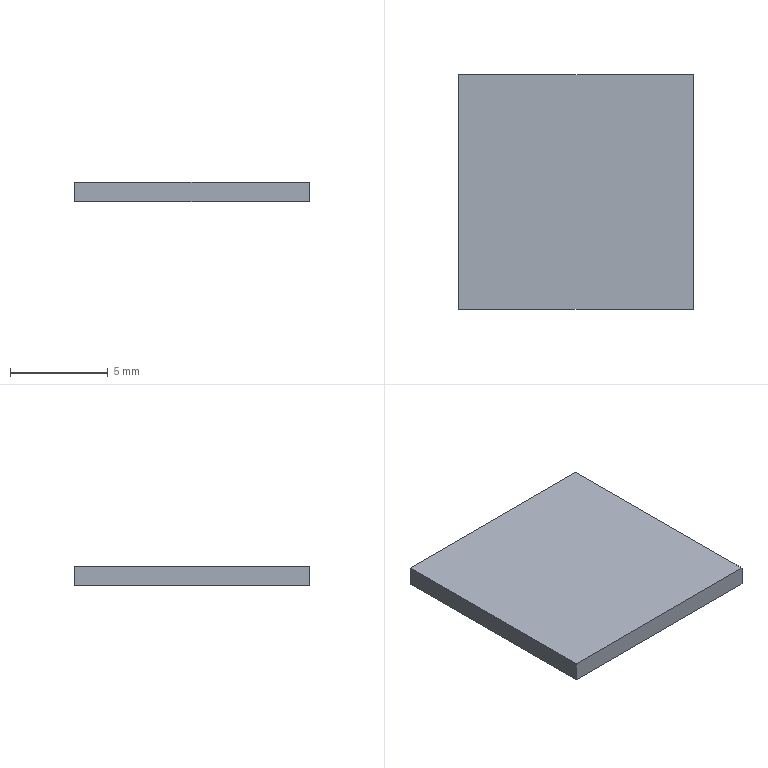Component | SolidWorks | 12x1x12WeldedSquare-1 | 1 solid | 6 faces | volume 144 mm3 | plane 6 | material 304